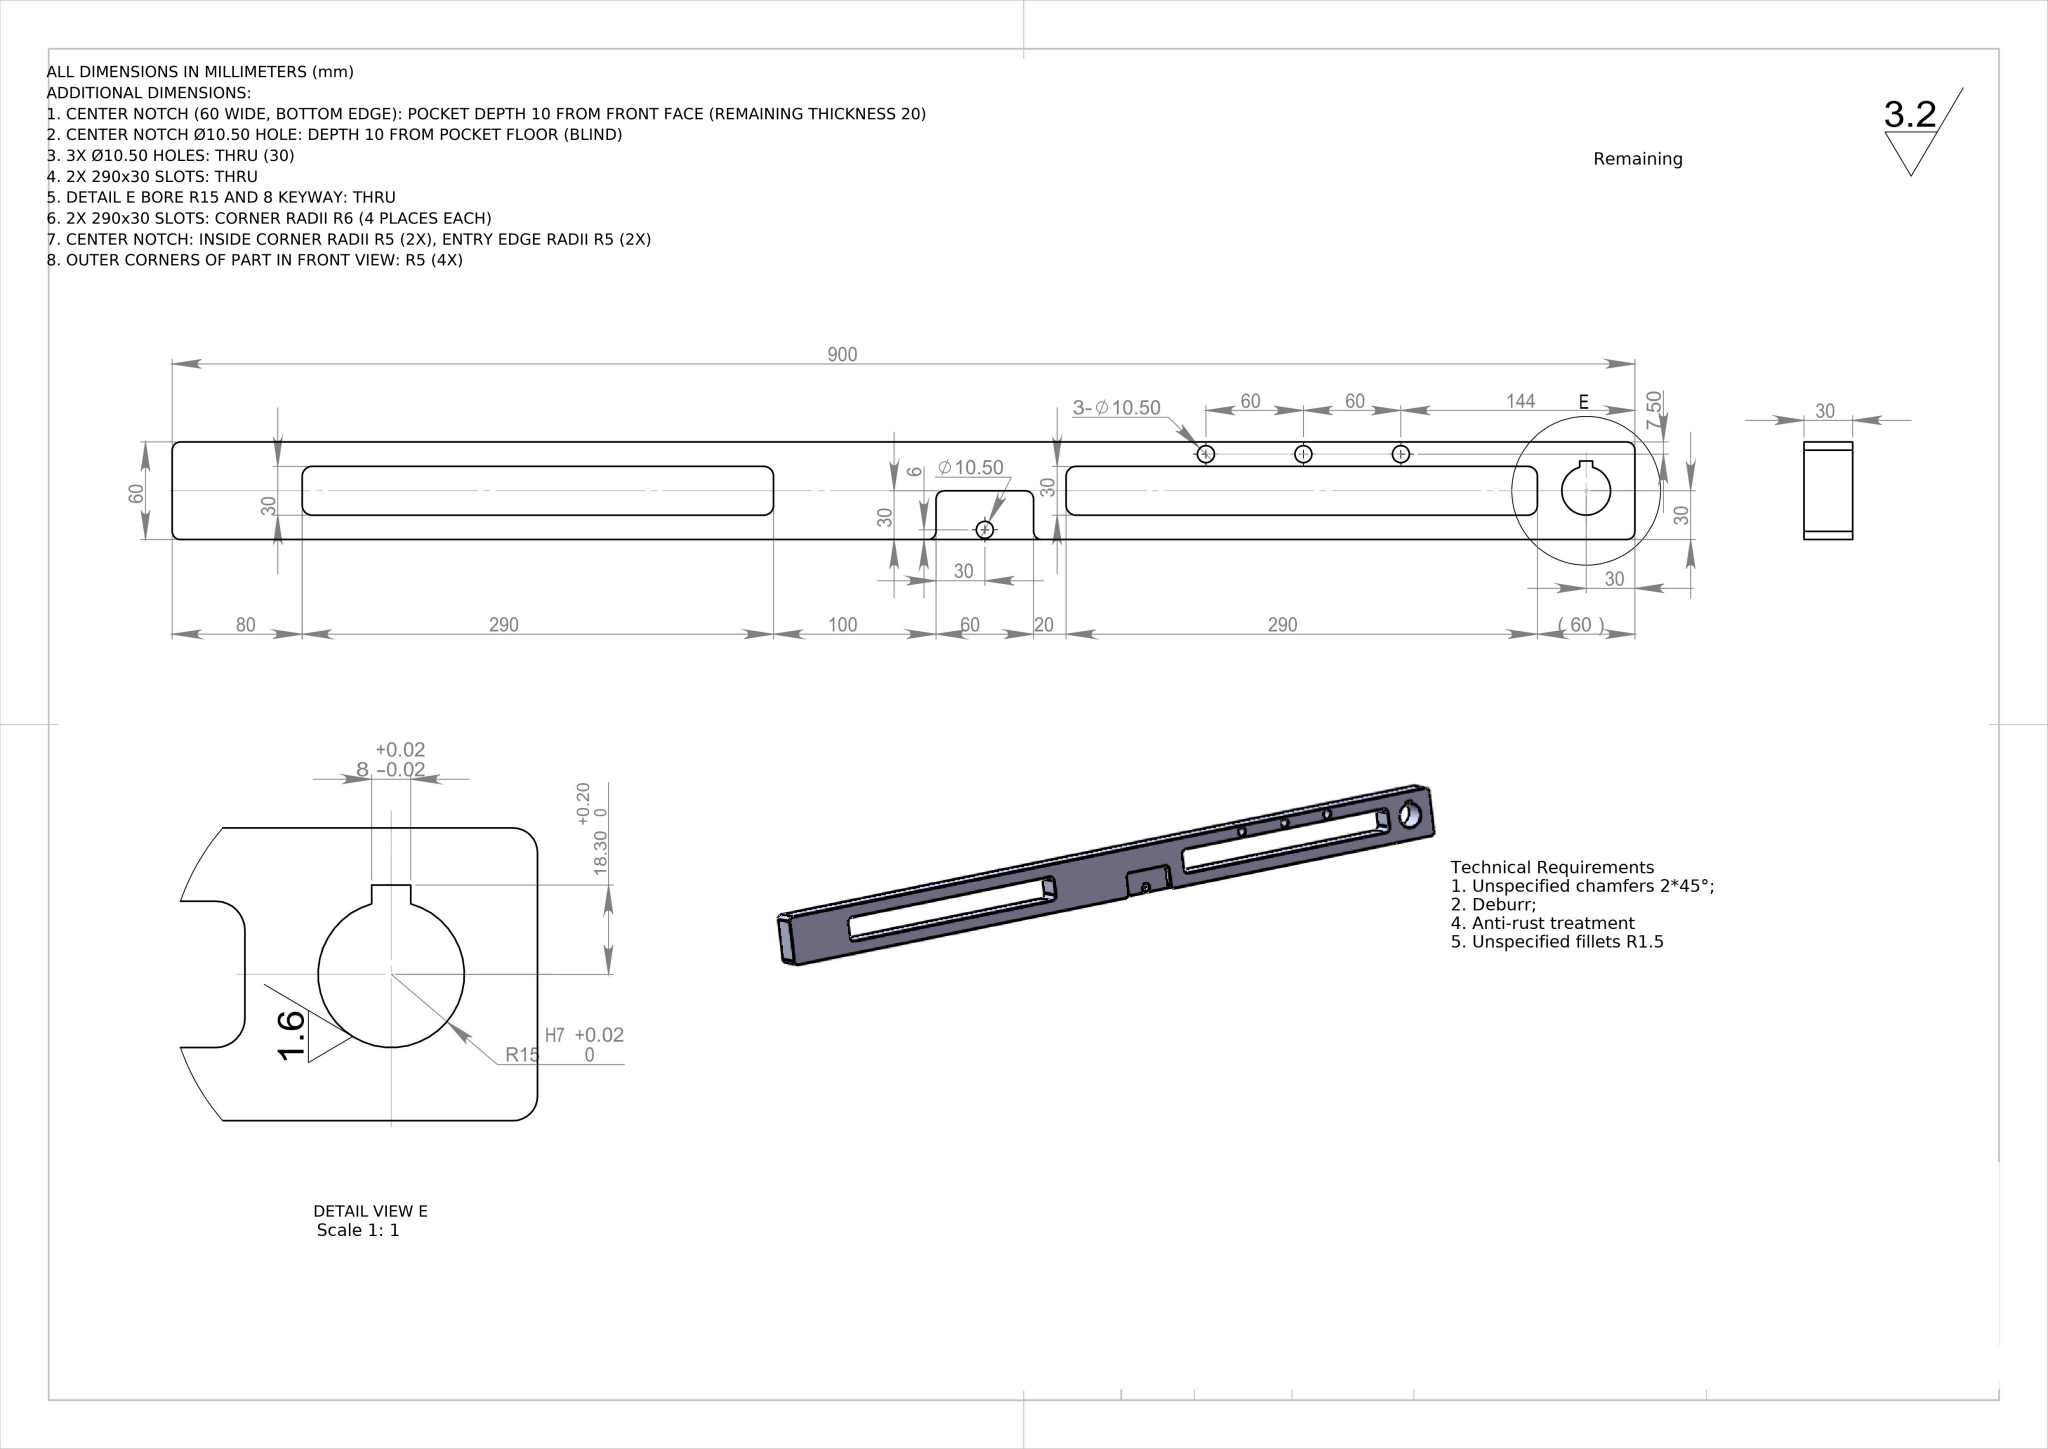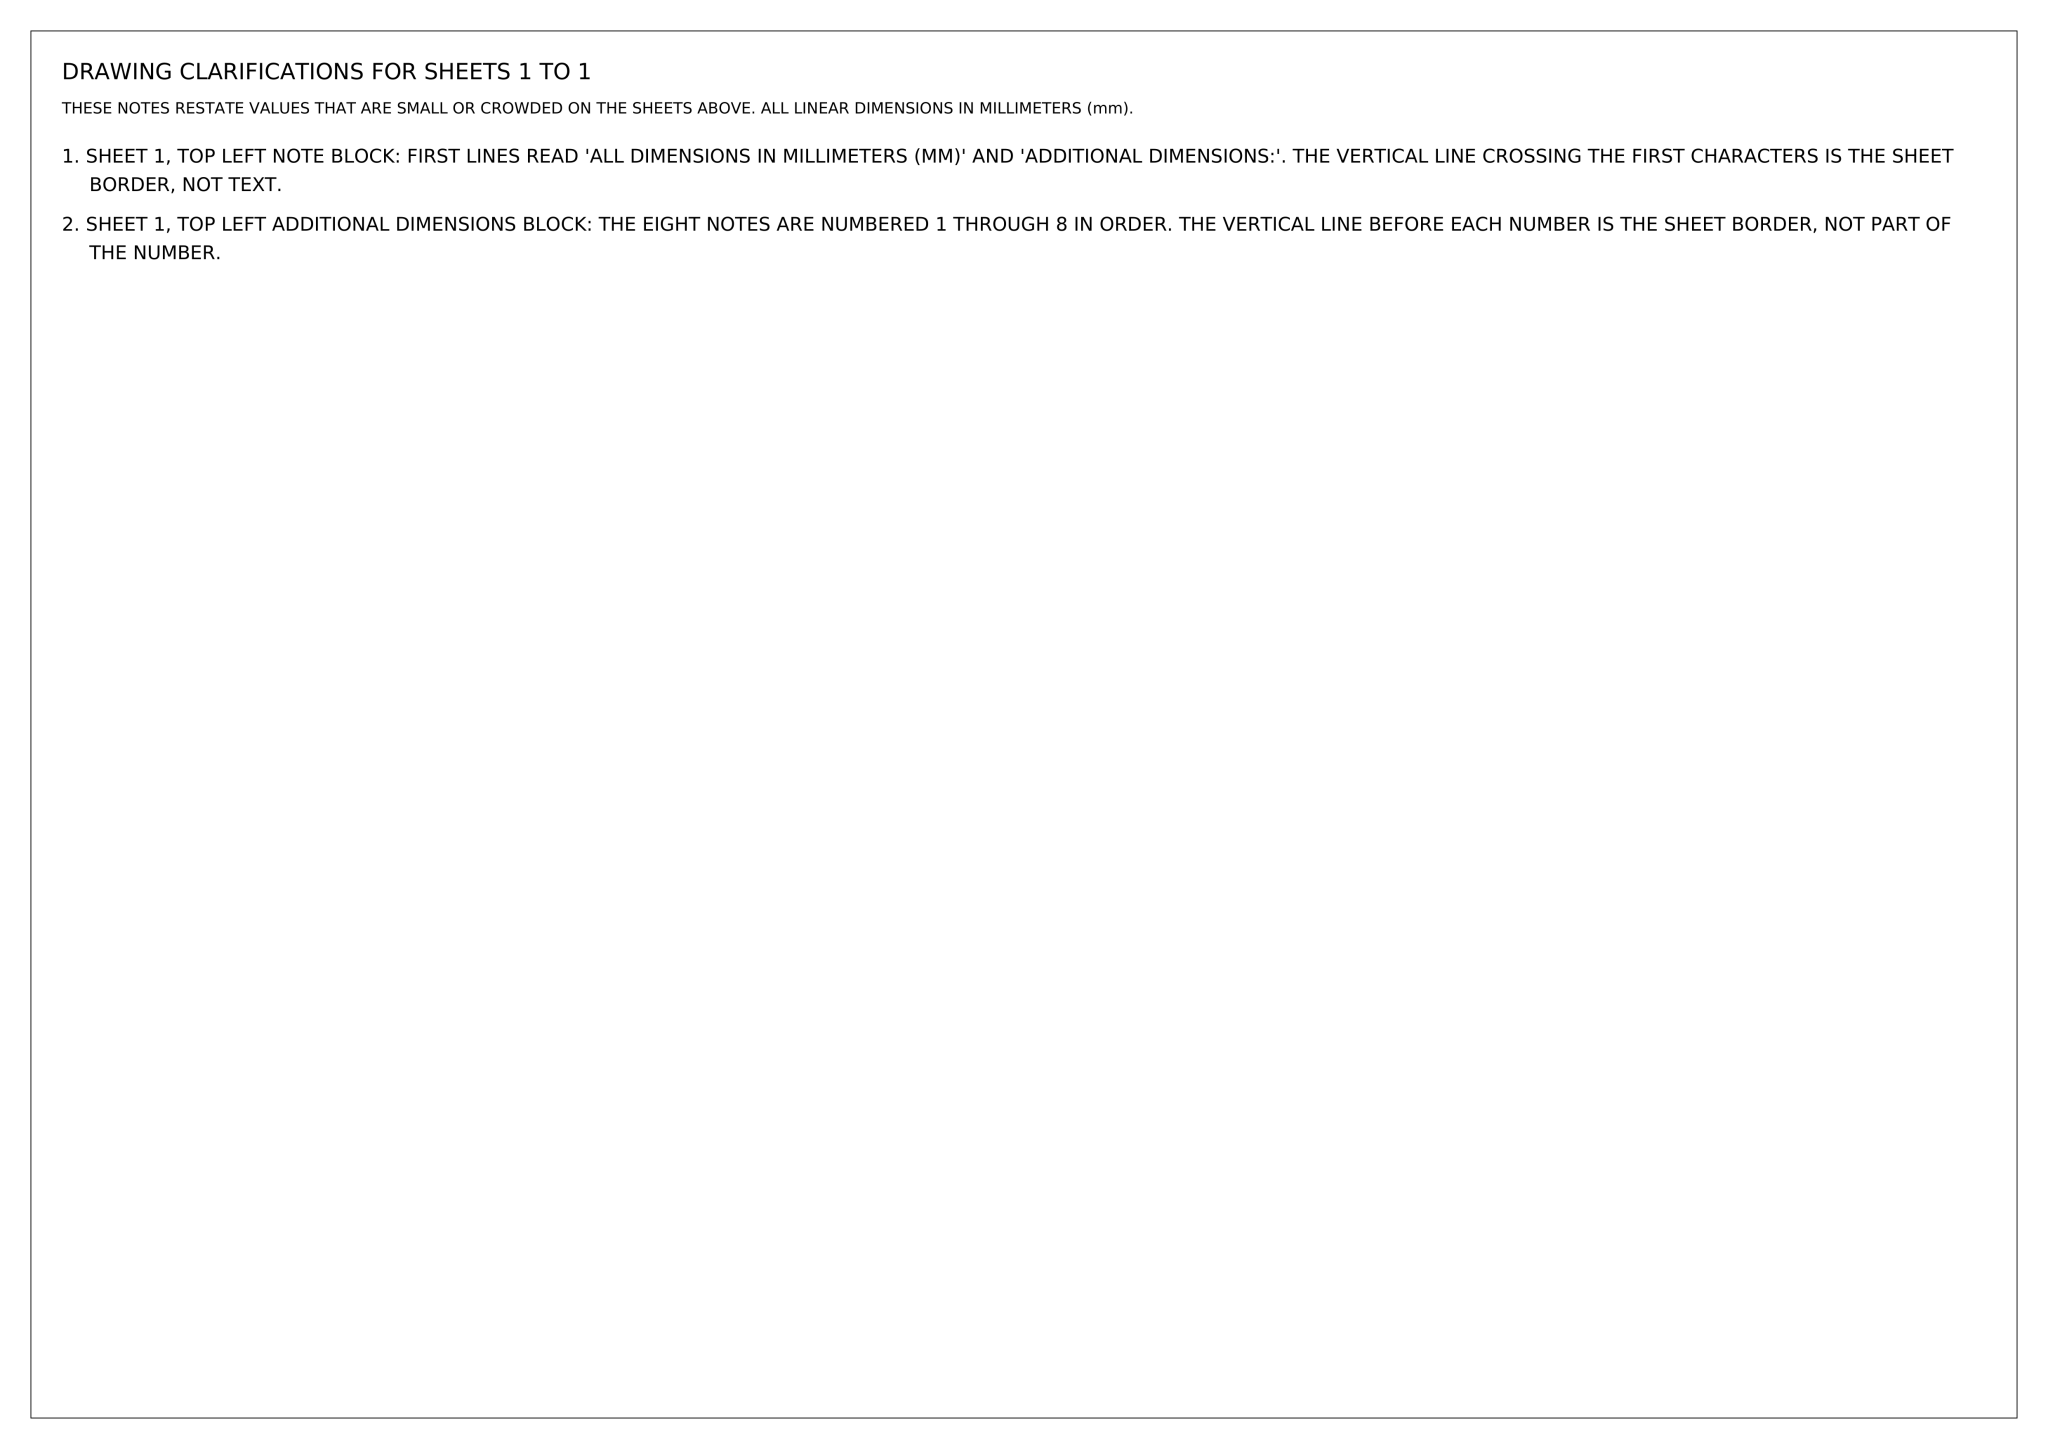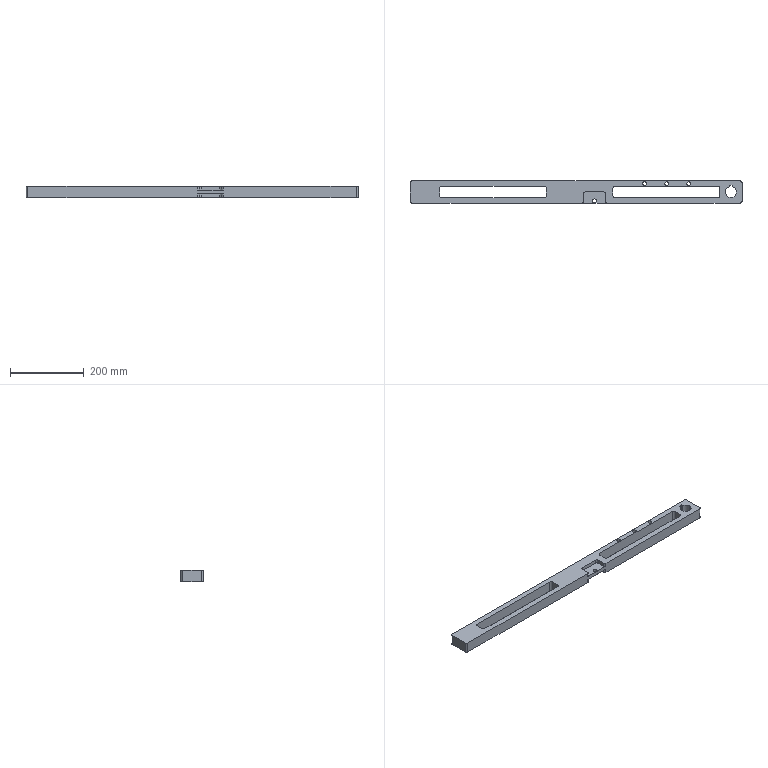Part | NX | mm | 1 solid | 56 faces | box 900 x 60 x 30 mm | volume 1032510 mm3 | cylinder 31 | plane 25 | commonest cylinder face diameters 10 x12 10.5 x8 12 x8 30 x3